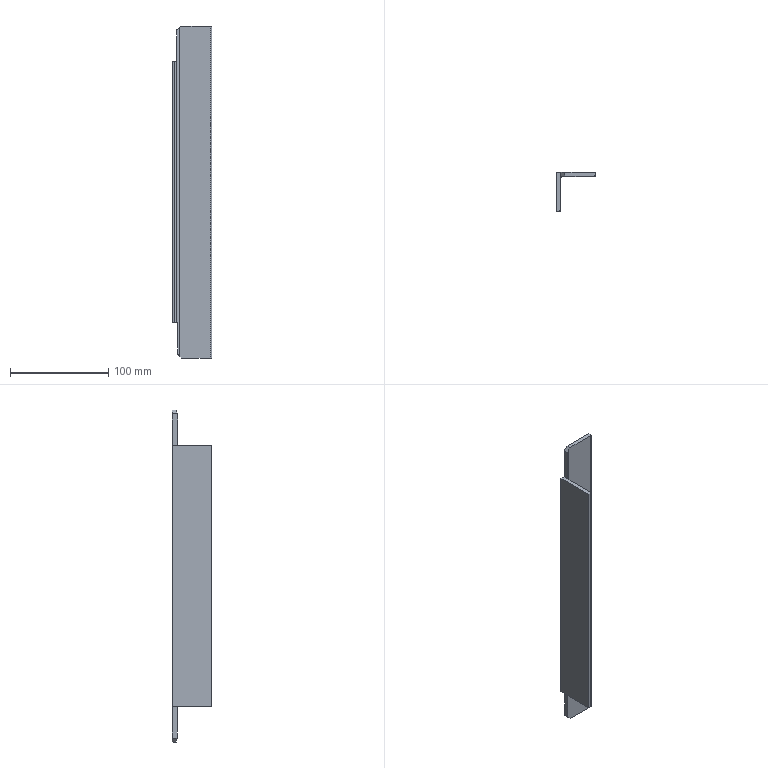Component | SolidWorks | FrameAssembly-1_LeftAndRightSideAngleSteel-1 | 1 solid | 17 faces | box 40 x 40 x 338 mm | volume 91426 mm3 | plane 14 | cylinder 3 | commonest cylinder face diameters 2.667 x2 7 x1
build123d program:
from build123d import *

# Parameters (mm, degrees)
BASE_DEPTH         = 338
SKETCH1_2_W        = 4.611
SKETCH1_2_H        = 42.038
CUT_EXTRUDE1_DEPTH = 36
SKETCH2_W          = 5.275
SKETCH2_H          = 47.654
CUT_EXTRUDE2_DEPTH = 36
CHAMFER1_SIZE      = 4


with BuildPart() as part:
    # Sketch1 → Base (new body)
    with BuildSketch(Plane.YZ):
        with BuildLine():
            Line((0, 40), (0, 0))
            Line((0, 0), (40, 0))
            Line((40, 0), (40, 2.667))
            ThreePointArc((40, 2.667), (39.609, 3.609), (38.667, 4))
            Line((38.667, 4), (7.5, 4))
            ThreePointArc((7.5, 4), (5.025, 5.025), (4, 7.5))
            Line((4, 7.5), (4, 38.667))
            ThreePointArc((4, 38.667), (3.609, 39.609), (2.667, 40))
            Line((2.667, 40), (0, 40))
        make_face()
    extrude(amount=BASE_DEPTH)

    # Sketch1_2 → Cut-Extrude1 (cut)
    with BuildSketch(Plane(origin=(338, 0, 0), x_dir=(0, 0, -1), z_dir=(1, 0, 0))):
        with Locations((-2.305, 18.981)):
            Rectangle(SKETCH1_2_W, SKETCH1_2_H)
    extrude(amount=-CUT_EXTRUDE1_DEPTH, mode=Mode.SUBTRACT)

    # Sketch2 → Cut-Extrude2 (cut)
    with BuildSketch(Plane.ZY):
        with Locations((2.637, 23.827)):
            Rectangle(SKETCH2_W, SKETCH2_H)
    extrude(amount=-CUT_EXTRUDE2_DEPTH, mode=Mode.SUBTRACT)

    # Chamfer1
    chamfer1_edges = [part.edges().sort_by_distance(p)[0] for p in [
        (338, 2.762, 4.611),
        (0, 2.399, 5.275),
    ]]
    chamfer(chamfer1_edges, length=CHAMFER1_SIZE)


solid = part.part

# Placed as in the assembly
solid = solid.moved(Location((-927.848, 492.395, 4), (180, 90, 0)))
STEP:
#1=COLOUR_RGB('',0.7922,0.8196,0.9333);
#2=FILL_AREA_STYLE_COLOUR('',#1);
#3=FILL_AREA_STYLE('',(#2));
#4=SURFACE_STYLE_FILL_AREA(#3);
#5=SURFACE_SIDE_STYLE('',(#4));
#6=SURFACE_STYLE_USAGE(.BOTH.,#5);
#7=PRESENTATION_STYLE_ASSIGNMENT((#6));
#8=CARTESIAN_POINT('',(-34.955,19.281,0.1575));
#9=VERTEX_POINT('',#8);
#10=CARTESIAN_POINT('',(-34.955,19.386,0.1575));
#11=VERTEX_POINT('',#10);
#12=CARTESIAN_POINT('',(-34.955,19.386,0.1575));
#13=DIRECTION('',(0.,1.,0.));
#14=VECTOR('',#13,39.37);
#15=LINE('',#12,#14);
#16=EDGE_CURVE('',#9,#11,#15,.T.);
#17=ORIENTED_EDGE('',*,*,#16,.T.);
#18=CARTESIAN_POINT('',(-34.955,19.386,13.465));
#19=VERTEX_POINT('',#18);
#20=CARTESIAN_POINT('',(-34.955,19.386,13.465));
#21=DIRECTION('',(-0.,0.,-1.));
#22=VECTOR('',#21,39.37);
#23=LINE('',#20,#22);
#24=EDGE_CURVE('',#19,#11,#23,.T.);
#25=ORIENTED_EDGE('',*,*,#24,.F.);
#26=CARTESIAN_POINT('',(-34.955,19.281,13.465));
#27=VERTEX_POINT('',#26);
#28=CARTESIAN_POINT('',(-34.955,19.386,13.465));
#29=DIRECTION('',(0.,1.,0.));
#30=VECTOR('',#29,39.37);
#31=LINE('',#28,#30);
#32=EDGE_CURVE('',#27,#19,#31,.T.);
#33=ORIENTED_EDGE('',*,*,#32,.F.);
#34=CARTESIAN_POINT('',(-34.955,19.281,13.465));
#35=DIRECTION('',(-0.,0.,-1.));
#36=VECTOR('',#35,39.37);
#37=LINE('',#34,#36);
#38=EDGE_CURVE('',#27,#9,#37,.T.);
#39=ORIENTED_EDGE('',*,*,#38,.T.);
#40=EDGE_LOOP('',(#17,#25,#33,#39));
#41=FACE_OUTER_BOUND('',#40,.T.);
#42=CARTESIAN_POINT('',(-34.955,19.386,13.465));
#43=DIRECTION('',(-1.,0.,0.));
#44=DIRECTION('',(-0.,0.,-1.));
#45=AXIS2_PLACEMENT_3D('',#42,#43,#44);
#46=PLANE('',#45);
#47=ADVANCED_FACE('',(#41),#46,.F.);
#48=CARTESIAN_POINT('',(-36.348,19.386,12.047));
#49=VERTEX_POINT('',#48);
#50=CARTESIAN_POINT('',(-36.348,19.386,13.307));
#51=VERTEX_POINT('',#50);
#52=CARTESIAN_POINT('',(-36.348,19.386,13.465));
#53=DIRECTION('',(0.,-0.,1.));
#54=VECTOR('',#53,39.37);
#55=LINE('',#52,#54);
#56=EDGE_CURVE('',#49,#51,#55,.T.);
#57=ORIENTED_EDGE('',*,*,#56,.T.);
#58=CARTESIAN_POINT('',(-36.19,19.386,13.465));
#59=VERTEX_POINT('',#58);
#60=CARTESIAN_POINT('',(-36.19,19.386,13.465));
#61=DIRECTION('',(0.7071,-0.,0.7071));
#62=VECTOR('',#61,39.37);
#63=LINE('',#60,#62);
#64=EDGE_CURVE('',#51,#59,#63,.T.);
#65=ORIENTED_EDGE('',*,*,#64,.T.);
#66=CARTESIAN_POINT('',(-34.955,19.386,13.465));
#67=DIRECTION('',(-1.,0.,0.));
#68=VECTOR('',#67,39.37);
#69=LINE('',#66,#68);
#70=EDGE_CURVE('',#19,#59,#69,.T.);
#71=ORIENTED_EDGE('',*,*,#70,.F.);
#72=ORIENTED_EDGE('',*,*,#24,.T.);
#73=CARTESIAN_POINT('',(-36.164,19.386,0.1575));
#74=VERTEX_POINT('',#73);
#75=CARTESIAN_POINT('',(-34.955,19.386,0.1575));
#76=DIRECTION('',(-1.,0.,0.));
#77=VECTOR('',#76,39.37);
#78=LINE('',#75,#77);
#79=EDGE_CURVE('',#11,#74,#78,.T.);
#80=ORIENTED_EDGE('',*,*,#79,.T.);
#81=CARTESIAN_POINT('',(-36.322,19.386,0.315));
#82=VERTEX_POINT('',#81);
#83=CARTESIAN_POINT('',(-36.322,19.386,0.315));
#84=DIRECTION('',(-0.7071,-0.,0.7071));
#85=VECTOR('',#84,39.37);
#86=LINE('',#83,#85);
#87=EDGE_CURVE('',#74,#82,#86,.T.);
#88=ORIENTED_EDGE('',*,*,#87,.T.);
#89=CARTESIAN_POINT('',(-36.322,19.386,1.575));
#90=VERTEX_POINT('',#89);
#91=CARTESIAN_POINT('',(-36.322,19.386,1.575));
#92=DIRECTION('',(-0.,0.,-1.));
#93=VECTOR('',#92,39.37);
#94=LINE('',#91,#93);
#95=EDGE_CURVE('',#90,#82,#94,.T.);
#96=ORIENTED_EDGE('',*,*,#95,.F.);
#97=CARTESIAN_POINT('',(-36.529,19.386,1.575));
#98=VERTEX_POINT('',#97);
#99=CARTESIAN_POINT('',(-36.529,19.386,1.575));
#100=DIRECTION('',(1.,-0.,-0.));
#101=VECTOR('',#100,39.37);
#102=LINE('',#99,#101);
#103=EDGE_CURVE('',#98,#90,#102,.T.);
#104=ORIENTED_EDGE('',*,*,#103,.F.);
#105=CARTESIAN_POINT('',(-36.529,19.386,12.047));
#106=VERTEX_POINT('',#105);
#107=CARTESIAN_POINT('',(-36.529,19.386,13.465));
#108=DIRECTION('',(-0.,0.,-1.));
#109=VECTOR('',#108,39.37);
#110=LINE('',#107,#109);
#111=EDGE_CURVE('',#106,#98,#110,.T.);
#112=ORIENTED_EDGE('',*,*,#111,.F.);
#113=CARTESIAN_POINT('',(-34.955,19.386,12.047));
#114=DIRECTION('',(1.,-0.,-0.));
#115=VECTOR('',#114,39.37);
#116=LINE('',#113,#115);
#117=EDGE_CURVE('',#106,#49,#116,.T.);
#118=ORIENTED_EDGE('',*,*,#117,.T.);
#119=EDGE_LOOP('',(#57,#65,#71,#72,#80,#88,#96,#104,#112,#118));
#120=FACE_OUTER_BOUND('',#119,.T.);
#121=CARTESIAN_POINT('',(-34.955,19.386,13.465));
#122=DIRECTION('',(-0.,-1.,-0.));
#123=DIRECTION('',(1.,-0.,-0.));
#124=AXIS2_PLACEMENT_3D('',#121,#122,#123);
#125=PLANE('',#124);
#126=ADVANCED_FACE('',(#120),#125,.F.);
#127=ORIENTED_EDGE('',*,*,#111,.T.);
#128=CARTESIAN_POINT('',(-36.529,17.811,1.575));
#129=VERTEX_POINT('',#128);
#130=CARTESIAN_POINT('',(-36.529,19.386,1.575));
#131=DIRECTION('',(0.,1.,0.));
#132=VECTOR('',#131,39.37);
#133=LINE('',#130,#132);
#134=EDGE_CURVE('',#129,#98,#133,.T.);
#135=ORIENTED_EDGE('',*,*,#134,.F.);
#136=CARTESIAN_POINT('',(-36.529,17.811,12.047));
#137=VERTEX_POINT('',#136);
#138=CARTESIAN_POINT('',(-36.529,17.811,13.465));
#139=DIRECTION('',(-0.,0.,-1.));
#140=VECTOR('',#139,39.37);
#141=LINE('',#138,#140);
#142=EDGE_CURVE('',#137,#129,#141,.T.);
#143=ORIENTED_EDGE('',*,*,#142,.F.);
#144=CARTESIAN_POINT('',(-36.529,17.811,12.047));
#145=DIRECTION('',(-0.,-1.,-0.));
#146=VECTOR('',#145,39.37);
#147=LINE('',#144,#146);
#148=EDGE_CURVE('',#106,#137,#147,.T.);
#149=ORIENTED_EDGE('',*,*,#148,.F.);
#150=EDGE_LOOP('',(#127,#135,#143,#149));
#151=FACE_OUTER_BOUND('',#150,.T.);
#152=CARTESIAN_POINT('',(-36.529,19.386,13.465));
#153=DIRECTION('',(1.,-0.,-0.));
#154=DIRECTION('',(0.,-0.,1.));
#155=AXIS2_PLACEMENT_3D('',#152,#153,#154);
#156=PLANE('',#155);
#157=ADVANCED_FACE('',(#151),#156,.F.);
#158=ORIENTED_EDGE('',*,*,#142,.T.);
#159=CARTESIAN_POINT('',(-36.424,17.811,1.575));
#160=VERTEX_POINT('',#159);
#161=CARTESIAN_POINT('',(-36.529,17.811,1.575));
#162=DIRECTION('',(1.,-0.,-0.));
#163=VECTOR('',#162,39.37);
#164=LINE('',#161,#163);
#165=EDGE_CURVE('',#129,#160,#164,.T.);
#166=ORIENTED_EDGE('',*,*,#165,.T.);
#167=CARTESIAN_POINT('',(-36.424,17.811,12.047));
#168=VERTEX_POINT('',#167);
#169=CARTESIAN_POINT('',(-36.424,17.811,13.465));
#170=DIRECTION('',(-0.,0.,-1.));
#171=VECTOR('',#170,39.37);
#172=LINE('',#169,#171);
#173=EDGE_CURVE('',#168,#160,#172,.T.);
#174=ORIENTED_EDGE('',*,*,#173,.F.);
#175=CARTESIAN_POINT('',(-36.529,17.811,12.047));
#176=DIRECTION('',(1.,-0.,-0.));
#177=VECTOR('',#176,39.37);
#178=LINE('',#175,#177);
#179=EDGE_CURVE('',#137,#168,#178,.T.);
#180=ORIENTED_EDGE('',*,*,#179,.F.);
#181=EDGE_LOOP('',(#158,#166,#174,#180));
#182=FACE_OUTER_BOUND('',#181,.T.);
#183=CARTESIAN_POINT('',(-36.529,17.811,13.465));
#184=DIRECTION('',(0.,1.,0.));
#185=DIRECTION('',(-1.,0.,0.));
#186=AXIS2_PLACEMENT_3D('',#183,#184,#185);
#187=PLANE('',#186);
#188=ADVANCED_FACE('',(#182),#187,.F.);
#189=ORIENTED_EDGE('',*,*,#173,.T.);
#190=CARTESIAN_POINT('',(-36.372,17.863,1.575));
#191=VERTEX_POINT('',#190);
#192=CARTESIAN_POINT('',(-36.424,17.863,1.575));
#193=DIRECTION('',(0.,-0.,1.));
#194=DIRECTION('',(-1.,0.,0.));
#195=AXIS2_PLACEMENT_3D('',#192,#193,#194);
#196=CIRCLE('',#195,0.05249);
#197=EDGE_CURVE('',#160,#191,#196,.T.);
#198=ORIENTED_EDGE('',*,*,#197,.T.);
#199=CARTESIAN_POINT('',(-36.372,17.863,12.047));
#200=VERTEX_POINT('',#199);
#201=CARTESIAN_POINT('',(-36.372,17.863,13.465));
#202=DIRECTION('',(-0.,0.,-1.));
#203=VECTOR('',#202,39.37);
#204=LINE('',#201,#203);
#205=EDGE_CURVE('',#200,#191,#204,.T.);
#206=ORIENTED_EDGE('',*,*,#205,.F.);
#207=CARTESIAN_POINT('',(-36.424,17.863,12.047));
#208=DIRECTION('',(-0.,0.,-1.));
#209=DIRECTION('',(1.,0.,0.));
#210=AXIS2_PLACEMENT_3D('',#207,#208,#209);
#211=CIRCLE('',#210,0.05249);
#212=EDGE_CURVE('',#200,#168,#211,.T.);
#213=ORIENTED_EDGE('',*,*,#212,.T.);
#214=EDGE_LOOP('',(#189,#198,#206,#213));
#215=FACE_OUTER_BOUND('',#214,.T.);
#216=CARTESIAN_POINT('',(-36.424,17.863,13.465));
#217=DIRECTION('',(-0.,0.,-1.));
#218=DIRECTION('',(1.,0.,0.));
#219=AXIS2_PLACEMENT_3D('',#216,#217,#218);
#220=CYLINDRICAL_SURFACE('',#219,0.05249);
#221=ADVANCED_FACE('',(#215),#220,.T.);
#222=ORIENTED_EDGE('',*,*,#205,.T.);
#223=CARTESIAN_POINT('',(-36.372,19.09,1.575));
#224=VERTEX_POINT('',#223);
#225=CARTESIAN_POINT('',(-36.372,19.09,1.575));
#226=DIRECTION('',(0.,1.,0.));
#227=VECTOR('',#226,39.37);
#228=LINE('',#225,#227);
#229=EDGE_CURVE('',#191,#224,#228,.T.);
#230=ORIENTED_EDGE('',*,*,#229,.T.);
#231=CARTESIAN_POINT('',(-36.372,19.09,12.047));
#232=VERTEX_POINT('',#231);
#233=CARTESIAN_POINT('',(-36.372,19.09,13.465));
#234=DIRECTION('',(-0.,0.,-1.));
#235=VECTOR('',#234,39.37);
#236=LINE('',#233,#235);
#237=EDGE_CURVE('',#232,#224,#236,.T.);
#238=ORIENTED_EDGE('',*,*,#237,.F.);
#239=CARTESIAN_POINT('',(-36.372,19.09,12.047));
#240=DIRECTION('',(-0.,-1.,-0.));
#241=VECTOR('',#240,39.37);
#242=LINE('',#239,#241);
#243=EDGE_CURVE('',#232,#200,#242,.T.);
#244=ORIENTED_EDGE('',*,*,#243,.T.);
#245=EDGE_LOOP('',(#222,#230,#238,#244));
#246=FACE_OUTER_BOUND('',#245,.T.);
#247=CARTESIAN_POINT('',(-36.372,19.09,13.465));
#248=DIRECTION('',(-1.,0.,0.));
#249=DIRECTION('',(-0.,0.,-1.));
#250=AXIS2_PLACEMENT_3D('',#247,#248,#249);
#251=PLANE('',#250);
#252=ADVANCED_FACE('',(#246),#251,.F.);
#253=CARTESIAN_POINT('',(-36.234,19.228,13.421));
#254=VERTEX_POINT('',#253);
#255=CARTESIAN_POINT('',(-36.234,19.228,0.2274));
#256=VERTEX_POINT('',#255);
#257=CARTESIAN_POINT('',(-36.234,19.228,13.465));
#258=DIRECTION('',(-0.,0.,-1.));
#259=VECTOR('',#258,39.37);
#260=LINE('',#257,#259);
#261=EDGE_CURVE('',#254,#256,#260,.T.);
#262=ORIENTED_EDGE('',*,*,#261,.F.);
#263=CARTESIAN_POINT('',(-36.348,19.168,13.307));
#264=VERTEX_POINT('',#263);
#265=CARTESIAN_POINT('',(-36.234,19.228,13.421));
#266=CARTESIAN_POINT('',(-36.281,19.228,13.374));
#267=CARTESIAN_POINT('',(-36.322,19.206,13.333));
#268=CARTESIAN_POINT('',(-36.348,19.168,13.307));
#269=(BOUNDED_CURVE()B_SPLINE_CURVE(3,(#265,#266,#267,#268),.UNSPECIFIED.,.F.,.F.)B_SPLINE_CURVE_WITH_KNOTS((4,4),(4.712,5.683),.UNSPECIFIED.)CURVE()GEOMETRIC_REPRESENTATION_ITEM()RATIONAL_B_SPLINE_CURVE((1.,0.923,0.923,1.))REPRESENTATION_ITEM(''));
#270=EDGE_CURVE('',#254,#264,#269,.T.);
#271=ORIENTED_EDGE('',*,*,#270,.T.);
#272=CARTESIAN_POINT('',(-36.348,19.168,12.047));
#273=VERTEX_POINT('',#272);
#274=CARTESIAN_POINT('',(-36.348,19.168,13.465));
#275=DIRECTION('',(-0.,0.,-1.));
#276=VECTOR('',#275,39.37);
#277=LINE('',#274,#276);
#278=EDGE_CURVE('',#264,#273,#277,.T.);
#279=ORIENTED_EDGE('',*,*,#278,.T.);
#280=CARTESIAN_POINT('',(-36.234,19.09,12.047));
#281=DIRECTION('',(0.,-0.,1.));
#282=DIRECTION('',(1.,-0.,0.));
#283=AXIS2_PLACEMENT_3D('',#280,#281,#282);
#284=CIRCLE('',#283,0.1378);
#285=EDGE_CURVE('',#273,#232,#284,.T.);
#286=ORIENTED_EDGE('',*,*,#285,.T.);
#287=ORIENTED_EDGE('',*,*,#237,.T.);
#288=CARTESIAN_POINT('',(-36.322,19.197,1.575));
#289=VERTEX_POINT('',#288);
#290=CARTESIAN_POINT('',(-36.234,19.09,1.575));
#291=DIRECTION('',(-0.,0.,-1.));
#292=DIRECTION('',(-1.,0.,0.));
#293=AXIS2_PLACEMENT_3D('',#290,#291,#292);
#294=CIRCLE('',#293,0.1378);
#295=EDGE_CURVE('',#224,#289,#294,.T.);
#296=ORIENTED_EDGE('',*,*,#295,.T.);
#297=CARTESIAN_POINT('',(-36.322,19.197,0.315));
#298=VERTEX_POINT('',#297);
#299=CARTESIAN_POINT('',(-36.322,19.197,13.465));
#300=DIRECTION('',(-0.,0.,-1.));
#301=VECTOR('',#300,39.37);
#302=LINE('',#299,#301);
#303=EDGE_CURVE('',#289,#298,#302,.T.);
#304=ORIENTED_EDGE('',*,*,#303,.T.);
#305=CARTESIAN_POINT('',(-36.322,19.197,0.315));
#306=CARTESIAN_POINT('',(-36.297,19.217,0.29));
#307=CARTESIAN_POINT('',(-36.266,19.228,0.2596));
#308=CARTESIAN_POINT('',(-36.234,19.228,0.2274));
#309=(BOUNDED_CURVE()B_SPLINE_CURVE(3,(#305,#306,#307,#308),.UNSPECIFIED.,.F.,.F.)B_SPLINE_CURVE_WITH_KNOTS((4,4),(4.023,4.712),.UNSPECIFIED.)CURVE()GEOMETRIC_REPRESENTATION_ITEM()RATIONAL_B_SPLINE_CURVE((1.,0.9608,0.9608,1.))REPRESENTATION_ITEM(''));
#310=EDGE_CURVE('',#298,#256,#309,.T.);
#311=ORIENTED_EDGE('',*,*,#310,.T.);
#312=EDGE_LOOP('',(#262,#271,#279,#286,#287,#296,#304,#311));
#313=FACE_OUTER_BOUND('',#312,.T.);
#314=CARTESIAN_POINT('',(-36.234,19.09,13.465));
#315=DIRECTION('',(-0.,0.,-1.));
#316=DIRECTION('',(1.,0.,0.));
#317=AXIS2_PLACEMENT_3D('',#314,#315,#316);
#318=CYLINDRICAL_SURFACE('',#317,0.1378);
#319=ADVANCED_FACE('',(#313),#318,.F.);
#320=CARTESIAN_POINT('',(-36.19,19.228,13.465));
#321=VERTEX_POINT('',#320);
#322=CARTESIAN_POINT('',(-35.007,19.228,13.465));
#323=VERTEX_POINT('',#322);
#324=CARTESIAN_POINT('',(-35.007,19.228,13.465));
#325=DIRECTION('',(1.,-0.,-0.));
#326=VECTOR('',#325,39.37);
#327=LINE('',#324,#326);
#328=EDGE_CURVE('',#321,#323,#327,.T.);
#329=ORIENTED_EDGE('',*,*,#328,.F.);
#330=CARTESIAN_POINT('',(-36.19,19.228,13.465));
#331=DIRECTION('',(-0.7071,0.,-0.7071));
#332=VECTOR('',#331,39.37);
#333=LINE('',#330,#332);
#334=EDGE_CURVE('',#321,#254,#333,.T.);
#335=ORIENTED_EDGE('',*,*,#334,.T.);
#336=ORIENTED_EDGE('',*,*,#261,.T.);
#337=CARTESIAN_POINT('',(-36.164,19.228,0.1575));
#338=VERTEX_POINT('',#337);
#339=CARTESIAN_POINT('',(-36.322,19.228,0.315));
#340=DIRECTION('',(0.7071,0.,-0.7071));
#341=VECTOR('',#340,39.37);
#342=LINE('',#339,#341);
#343=EDGE_CURVE('',#256,#338,#342,.T.);
#344=ORIENTED_EDGE('',*,*,#343,.T.);
#345=CARTESIAN_POINT('',(-35.007,19.228,0.1575));
#346=VERTEX_POINT('',#345);
#347=CARTESIAN_POINT('',(-35.007,19.228,0.1575));
#348=DIRECTION('',(1.,-0.,-0.));
#349=VECTOR('',#348,39.37);
#350=LINE('',#347,#349);
#351=EDGE_CURVE('',#338,#346,#350,.T.);
#352=ORIENTED_EDGE('',*,*,#351,.T.);
#353=CARTESIAN_POINT('',(-35.007,19.228,13.465));
#354=DIRECTION('',(-0.,0.,-1.));
#355=VECTOR('',#354,39.37);
#356=LINE('',#353,#355);
#357=EDGE_CURVE('',#323,#346,#356,.T.);
#358=ORIENTED_EDGE('',*,*,#357,.F.);
#359=EDGE_LOOP('',(#329,#335,#336,#344,#352,#358));
#360=FACE_OUTER_BOUND('',#359,.T.);
#361=CARTESIAN_POINT('',(-35.007,19.228,13.465));
#362=DIRECTION('',(0.,1.,0.));
#363=DIRECTION('',(-1.,0.,0.));
#364=AXIS2_PLACEMENT_3D('',#361,#362,#363);
#365=PLANE('',#364);
#366=ADVANCED_FACE('',(#360),#365,.F.);
#367=CARTESIAN_POINT('',(-35.007,19.281,0.1575));
#368=DIRECTION('',(0.,-0.,1.));
#369=DIRECTION('',(1.,0.,0.));
#370=AXIS2_PLACEMENT_3D('',#367,#368,#369);
#371=CIRCLE('',#370,0.05249);
#372=EDGE_CURVE('',#346,#9,#371,.T.);
#373=ORIENTED_EDGE('',*,*,#372,.T.);
#374=ORIENTED_EDGE('',*,*,#38,.F.);
#375=CARTESIAN_POINT('',(-35.007,19.281,13.465));
#376=DIRECTION('',(0.,-0.,1.));
#377=DIRECTION('',(1.,0.,0.));
#378=AXIS2_PLACEMENT_3D('',#375,#376,#377);
#379=CIRCLE('',#378,0.05249);
#380=EDGE_CURVE('',#323,#27,#379,.T.);
#381=ORIENTED_EDGE('',*,*,#380,.F.);
#382=ORIENTED_EDGE('',*,*,#357,.T.);
#383=EDGE_LOOP('',(#373,#374,#381,#382));
#384=FACE_OUTER_BOUND('',#383,.T.);
#385=CARTESIAN_POINT('',(-35.007,19.281,13.465));
#386=DIRECTION('',(-0.,0.,-1.));
#387=DIRECTION('',(1.,0.,0.));
#388=AXIS2_PLACEMENT_3D('',#385,#386,#387);
#389=CYLINDRICAL_SURFACE('',#388,0.05249);
#390=ADVANCED_FACE('',(#384),#389,.T.);
#391=ORIENTED_EDGE('',*,*,#70,.T.);
#392=CARTESIAN_POINT('',(-36.19,19.281,13.465));
#393=DIRECTION('',(-0.,-1.,-0.));
#394=VECTOR('',#393,39.37);
#395=LINE('',#392,#394);
#396=EDGE_CURVE('',#59,#321,#395,.T.);
#397=ORIENTED_EDGE('',*,*,#396,.T.);
#398=ORIENTED_EDGE('',*,*,#328,.T.);
#399=ORIENTED_EDGE('',*,*,#380,.T.);
#400=ORIENTED_EDGE('',*,*,#32,.T.);
#401=EDGE_LOOP('',(#391,#397,#398,#399,#400));
#402=FACE_OUTER_BOUND('',#401,.T.);
#403=CARTESIAN_POINT('',(-35.007,19.281,13.465));
#404=DIRECTION('',(-0.,0.,-1.));
#405=DIRECTION('',(1.,-0.,-0.));
#406=AXIS2_PLACEMENT_3D('',#403,#404,#405);
#407=PLANE('',#406);
#408=ADVANCED_FACE('',(#402),#407,.F.);
#409=ORIENTED_EDGE('',*,*,#351,.F.);
#410=CARTESIAN_POINT('',(-36.164,19.386,0.1575));
#411=DIRECTION('',(0.,1.,0.));
#412=VECTOR('',#411,39.37);
#413=LINE('',#410,#412);
#414=EDGE_CURVE('',#338,#74,#413,.T.);
#415=ORIENTED_EDGE('',*,*,#414,.T.);
#416=ORIENTED_EDGE('',*,*,#79,.F.);
#417=ORIENTED_EDGE('',*,*,#16,.F.);
#418=ORIENTED_EDGE('',*,*,#372,.F.);
#419=EDGE_LOOP('',(#409,#415,#416,#417,#418));
#420=FACE_OUTER_BOUND('',#419,.T.);
#421=CARTESIAN_POINT('',(-35.007,19.281,0.1575));
#422=DIRECTION('',(-0.,0.,-1.));
#423=DIRECTION('',(1.,-0.,-0.));
#424=AXIS2_PLACEMENT_3D('',#421,#422,#423);
#425=PLANE('',#424);
#426=ADVANCED_FACE('',(#420),#425,.T.);
#427=ORIENTED_EDGE('',*,*,#148,.T.);
#428=ORIENTED_EDGE('',*,*,#179,.T.);
#429=ORIENTED_EDGE('',*,*,#212,.F.);
#430=ORIENTED_EDGE('',*,*,#243,.F.);
#431=ORIENTED_EDGE('',*,*,#285,.F.);
#432=CARTESIAN_POINT('',(-36.348,17.811,12.047));
#433=DIRECTION('',(0.,1.,0.));
#434=VECTOR('',#433,39.37);
#435=LINE('',#432,#434);
#436=EDGE_CURVE('',#273,#49,#435,.T.);
#437=ORIENTED_EDGE('',*,*,#436,.T.);
#438=ORIENTED_EDGE('',*,*,#117,.F.);
#439=EDGE_LOOP('',(#427,#428,#429,#430,#431,#437,#438));
#440=FACE_OUTER_BOUND('',#439,.T.);
#441=CARTESIAN_POINT('',(-36.529,19.466,12.047));
#442=DIRECTION('',(-0.,0.,-1.));
#443=DIRECTION('',(1.,-0.,-0.));
#444=AXIS2_PLACEMENT_3D('',#441,#442,#443);
#445=PLANE('',#444);
#446=ADVANCED_FACE('',(#440),#445,.F.);
#447=ORIENTED_EDGE('',*,*,#278,.F.);
#448=CARTESIAN_POINT('',(-36.348,17.811,13.307));
#449=DIRECTION('',(0.,1.,0.));
#450=VECTOR('',#449,39.37);
#451=LINE('',#448,#450);
#452=EDGE_CURVE('',#264,#51,#451,.T.);
#453=ORIENTED_EDGE('',*,*,#452,.T.);
#454=ORIENTED_EDGE('',*,*,#56,.F.);
#455=ORIENTED_EDGE('',*,*,#436,.F.);
#456=EDGE_LOOP('',(#447,#453,#454,#455));
#457=FACE_OUTER_BOUND('',#456,.T.);
#458=CARTESIAN_POINT('',(-36.348,17.811,12.047));
#459=DIRECTION('',(1.,-0.,-0.));
#460=DIRECTION('',(0.,-0.,1.));
#461=AXIS2_PLACEMENT_3D('',#458,#459,#460);
#462=PLANE('',#461);
#463=ADVANCED_FACE('',(#457),#462,.F.);
#464=ORIENTED_EDGE('',*,*,#134,.T.);
#465=ORIENTED_EDGE('',*,*,#103,.T.);
#466=CARTESIAN_POINT('',(-36.322,19.386,1.575));
#467=DIRECTION('',(-0.,-1.,-0.));
#468=VECTOR('',#467,39.37);
#469=LINE('',#466,#468);
#470=EDGE_CURVE('',#90,#289,#469,.T.);
#471=ORIENTED_EDGE('',*,*,#470,.T.);
#472=ORIENTED_EDGE('',*,*,#295,.F.);
#473=ORIENTED_EDGE('',*,*,#229,.F.);
#474=ORIENTED_EDGE('',*,*,#197,.F.);
#475=ORIENTED_EDGE('',*,*,#165,.F.);
#476=EDGE_LOOP('',(#464,#465,#471,#472,#473,#474,#475));
#477=FACE_OUTER_BOUND('',#476,.T.);
#478=CARTESIAN_POINT('',(-36.529,17.51,1.575));
#479=DIRECTION('',(0.,-0.,1.));
#480=DIRECTION('',(-1.,0.,0.));
#481=AXIS2_PLACEMENT_3D('',#478,#479,#480);
#482=PLANE('',#481);
#483=ADVANCED_FACE('',(#477),#482,.F.);
#484=ORIENTED_EDGE('',*,*,#95,.T.);
#485=CARTESIAN_POINT('',(-36.322,19.197,0.315));
#486=DIRECTION('',(-0.,-1.,-0.));
#487=VECTOR('',#486,39.37);
#488=LINE('',#485,#487);
#489=EDGE_CURVE('',#82,#298,#488,.T.);
#490=ORIENTED_EDGE('',*,*,#489,.T.);
#491=ORIENTED_EDGE('',*,*,#303,.F.);
#492=ORIENTED_EDGE('',*,*,#470,.F.);
#493=EDGE_LOOP('',(#484,#490,#491,#492));
#494=FACE_OUTER_BOUND('',#493,.T.);
#495=CARTESIAN_POINT('',(-36.322,19.386,1.575));
#496=DIRECTION('',(1.,-0.,-0.));
#497=DIRECTION('',(0.,-0.,1.));
#498=AXIS2_PLACEMENT_3D('',#495,#496,#497);
#499=PLANE('',#498);
#500=ADVANCED_FACE('',(#494),#499,.F.);
#501=ORIENTED_EDGE('',*,*,#64,.F.);
#502=ORIENTED_EDGE('',*,*,#452,.F.);
#503=ORIENTED_EDGE('',*,*,#270,.F.);
#504=ORIENTED_EDGE('',*,*,#334,.F.);
#505=ORIENTED_EDGE('',*,*,#396,.F.);
#506=EDGE_LOOP('',(#501,#502,#503,#504,#505));
#507=FACE_OUTER_BOUND('',#506,.T.);
#508=CARTESIAN_POINT('',(-36.19,19.281,13.465));
#509=DIRECTION('',(0.7071,0.,-0.7071));
#510=DIRECTION('',(0.7071,-0.,0.7071));
#511=AXIS2_PLACEMENT_3D('',#508,#509,#510);
#512=PLANE('',#511);
#513=ADVANCED_FACE('',(#507),#512,.F.);
#514=ORIENTED_EDGE('',*,*,#87,.F.);
#515=ORIENTED_EDGE('',*,*,#414,.F.);
#516=ORIENTED_EDGE('',*,*,#343,.F.);
#517=ORIENTED_EDGE('',*,*,#310,.F.);
#518=ORIENTED_EDGE('',*,*,#489,.F.);
#519=EDGE_LOOP('',(#514,#515,#516,#517,#518));
#520=FACE_OUTER_BOUND('',#519,.T.);
#521=CARTESIAN_POINT('',(-36.322,19.386,0.315));
#522=DIRECTION('',(-0.7071,0.,-0.7071));
#523=DIRECTION('',(0.7071,0.,-0.7071));
#524=AXIS2_PLACEMENT_3D('',#521,#522,#523);
#525=PLANE('',#524);
#526=ADVANCED_FACE('',(#520),#525,.T.);
#527=CLOSED_SHELL('',(#47,#126,#157,#188,#221,#252,#319,#366,#390,#408,#426,#446,#463,#483,#500,#513,#526));
#528=MANIFOLD_SOLID_BREP('',#527);
#529=STYLED_ITEM('',(#7),#528);
#530=(LENGTH_UNIT()NAMED_UNIT(*)SI_UNIT($,.METRE.));
#531=LENGTH_MEASURE_WITH_UNIT(LENGTH_MEASURE(0.0254),#530);
#532=DIMENSIONAL_EXPONENTS(1.,0.,0.,0.,0.,0.,0.);
#533=(CONVERSION_BASED_UNIT('',#531)LENGTH_UNIT()NAMED_UNIT(#532));
#534=UNCERTAINTY_MEASURE_WITH_UNIT(LENGTH_MEASURE(0.00001),#533,'','');
#535=(NAMED_UNIT(*)PLANE_ANGLE_UNIT()SI_UNIT($,.RADIAN.));
#536=(NAMED_UNIT(*)SI_UNIT($,.STERADIAN.)SOLID_ANGLE_UNIT());
#537=(GEOMETRIC_REPRESENTATION_CONTEXT(3)GLOBAL_UNCERTAINTY_ASSIGNED_CONTEXT((#534))GLOBAL_UNIT_ASSIGNED_CONTEXT((#533,#535,#536))REPRESENTATION_CONTEXT('',''));
#538=MECHANICAL_DESIGN_GEOMETRIC_PRESENTATION_REPRESENTATION('',(#529),#537);
#539=CARTESIAN_POINT('',(0.,0.,0.));
#540=DIRECTION('',(0.,0.,1.));
#541=DIRECTION('',(1.,0.,0.));
#542=AXIS2_PLACEMENT_3D('',#539,#540,#541);
#543=(LENGTH_UNIT()NAMED_UNIT(*)SI_UNIT($,.METRE.));
#544=LENGTH_MEASURE_WITH_UNIT(LENGTH_MEASURE(0.0254),#543);
#545=DIMENSIONAL_EXPONENTS(1.,0.,0.,0.,0.,0.,0.);
#546=(CONVERSION_BASED_UNIT('',#544)LENGTH_UNIT()NAMED_UNIT(#545));
#547=UNCERTAINTY_MEASURE_WITH_UNIT(LENGTH_MEASURE(0.00001),#546,'','');
#548=(NAMED_UNIT(*)PLANE_ANGLE_UNIT()SI_UNIT($,.RADIAN.));
#549=(NAMED_UNIT(*)SI_UNIT($,.STERADIAN.)SOLID_ANGLE_UNIT());
#550=(GEOMETRIC_REPRESENTATION_CONTEXT(3)GLOBAL_UNCERTAINTY_ASSIGNED_CONTEXT((#547))GLOBAL_UNIT_ASSIGNED_CONTEXT((#546,#548,#549))REPRESENTATION_CONTEXT('',''));
#551=ADVANCED_BREP_SHAPE_REPRESENTATION('',(#528,#542),#550);
#552=PRESENTATION_LAYER_ASSIGNMENT('','',(#529));